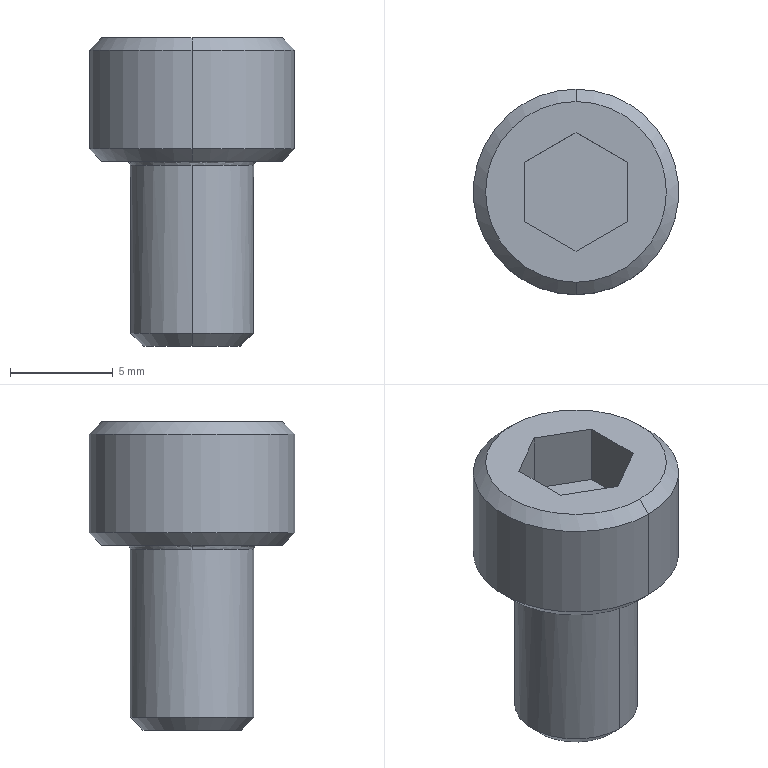Component | SolidWorks | TR-20x75-S-GN-1 (0)-3_5-1 | 1 solid | 22 faces | box 10 x 10 x 15 mm | volume 647 mm3 | plane 10 | cone 6 | cylinder 4 | spline 2 | commonest cylinder face diameters 6 x2 10 x2
STEP:
#1=COLOUR_RGB('',0.7922,0.8196,0.9333);
#2=FILL_AREA_STYLE_COLOUR('',#1);
#3=FILL_AREA_STYLE('',(#2));
#4=SURFACE_STYLE_FILL_AREA(#3);
#5=SURFACE_SIDE_STYLE('',(#4));
#6=SURFACE_STYLE_USAGE(.BOTH.,#5);
#7=PRESENTATION_STYLE_ASSIGNMENT((#6));
#8=CARTESIAN_POINT('',(7.52,25.197,0.4055));
#9=VERTEX_POINT('',#8);
#10=CARTESIAN_POINT('',(7.638,25.315,0.4055));
#11=VERTEX_POINT('',#10);
#12=CARTESIAN_POINT('',(7.638,25.197,0.4055));
#13=DIRECTION('',(-0.,0.,-1.));
#14=DIRECTION('',(0.,-1.,-0.));
#15=AXIS2_PLACEMENT_3D('',#12,#13,#14);
#16=CIRCLE('',#15,0.1181);
#17=EDGE_CURVE('',#9,#11,#16,.T.);
#18=ORIENTED_EDGE('',*,*,#17,.F.);
#19=CARTESIAN_POINT('',(7.512,25.197,0.4134));
#20=VERTEX_POINT('',#19);
#21=CARTESIAN_POINT('',(7.512,25.197,0.4055));
#22=DIRECTION('',(-0.,-1.,-0.));
#23=DIRECTION('',(-1.,0.,0.));
#24=AXIS2_PLACEMENT_3D('',#21,#22,#23);
#25=CIRCLE('',#24,0.007874);
#26=EDGE_CURVE('',#9,#20,#25,.T.);
#27=ORIENTED_EDGE('',*,*,#26,.T.);
#28=CARTESIAN_POINT('',(7.638,25.323,0.4134));
#29=VERTEX_POINT('',#28);
#30=CARTESIAN_POINT('',(7.638,25.323,0.4134));
#31=CARTESIAN_POINT('',(7.63,25.323,0.4134));
#32=CARTESIAN_POINT('',(7.618,25.322,0.4134));
#33=CARTESIAN_POINT('',(7.605,25.319,0.4134));
#34=CARTESIAN_POINT('',(7.598,25.316,0.4134));
#35=CARTESIAN_POINT('',(7.595,25.315,0.4134));
#36=CARTESIAN_POINT('',(7.593,25.315,0.4134));
#37=CARTESIAN_POINT('',(7.592,25.314,0.4134));
#38=CARTESIAN_POINT('',(7.575,25.308,0.4134));
#39=CARTESIAN_POINT('',(7.561,25.298,0.4134));
#40=CARTESIAN_POINT('',(7.543,25.28,0.4134));
#41=CARTESIAN_POINT('',(7.534,25.27,0.4134));
#42=CARTESIAN_POINT('',(7.527,25.257,0.4134));
#43=CARTESIAN_POINT('',(7.524,25.25,0.4134));
#44=CARTESIAN_POINT('',(7.522,25.247,0.4134));
#45=CARTESIAN_POINT('',(7.521,25.245,0.4134));
#46=CARTESIAN_POINT('',(7.521,25.244,0.4134));
#47=CARTESIAN_POINT('',(7.515,25.228,0.4134));
#48=CARTESIAN_POINT('',(7.512,25.213,0.4134));
#49=CARTESIAN_POINT('',(7.512,25.197,0.4134));
#50=B_SPLINE_CURVE_WITH_KNOTS('',3,(#30,#31,#32,#33,#34,#35,#36,#37,#38,#39,#40,#41,#42,#43,#44,#45,#46,#47,#48,#49),.UNSPECIFIED.,.F.,.F.,(4,1,1,1,2,2,2,1,1,1,2,2,4),(0.,0.125,0.1875,0.2188,0.2344,0.25,0.5,0.625,0.6875,0.7188,0.7344,0.75,1.),.UNSPECIFIED.);
#51=EDGE_CURVE('',#29,#20,#50,.T.);
#52=ORIENTED_EDGE('',*,*,#51,.F.);
#53=CARTESIAN_POINT('',(7.764,25.197,0.4134));
#54=VERTEX_POINT('',#53);
#55=CARTESIAN_POINT('',(7.764,25.197,0.4134));
#56=CARTESIAN_POINT('',(7.764,25.205,0.4134));
#57=CARTESIAN_POINT('',(7.763,25.217,0.4134));
#58=CARTESIAN_POINT('',(7.759,25.23,0.4134));
#59=CARTESIAN_POINT('',(7.757,25.237,0.4134));
#60=CARTESIAN_POINT('',(7.756,25.239,0.4134));
#61=CARTESIAN_POINT('',(7.756,25.241,0.4134));
#62=CARTESIAN_POINT('',(7.755,25.242,0.4134));
#63=CARTESIAN_POINT('',(7.749,25.259,0.4134));
#64=CARTESIAN_POINT('',(7.739,25.274,0.4134));
#65=CARTESIAN_POINT('',(7.721,25.292,0.4134));
#66=CARTESIAN_POINT('',(7.711,25.3,0.4134));
#67=CARTESIAN_POINT('',(7.698,25.308,0.4134));
#68=CARTESIAN_POINT('',(7.691,25.311,0.4134));
#69=CARTESIAN_POINT('',(7.688,25.312,0.4134));
#70=CARTESIAN_POINT('',(7.686,25.313,0.4134));
#71=CARTESIAN_POINT('',(7.685,25.314,0.4134));
#72=CARTESIAN_POINT('',(7.669,25.32,0.4134));
#73=CARTESIAN_POINT('',(7.654,25.323,0.4134));
#74=CARTESIAN_POINT('',(7.638,25.323,0.4134));
#75=B_SPLINE_CURVE_WITH_KNOTS('',3,(#55,#56,#57,#58,#59,#60,#61,#62,#63,#64,#65,#66,#67,#68,#69,#70,#71,#72,#73,#74),.UNSPECIFIED.,.F.,.F.,(4,1,1,1,2,2,2,1,1,1,2,2,4),(0.,0.125,0.1875,0.2187,0.2344,0.25,0.5,0.625,0.6875,0.7188,0.7344,0.75,1.),.UNSPECIFIED.);
#76=EDGE_CURVE('',#54,#29,#75,.T.);
#77=ORIENTED_EDGE('',*,*,#76,.F.);
#78=CARTESIAN_POINT('',(7.756,25.197,0.4055));
#79=VERTEX_POINT('',#78);
#80=CARTESIAN_POINT('',(7.764,25.197,0.4055));
#81=DIRECTION('',(0.,1.,0.));
#82=DIRECTION('',(1.,0.,0.));
#83=AXIS2_PLACEMENT_3D('',#80,#81,#82);
#84=CIRCLE('',#83,0.007874);
#85=EDGE_CURVE('',#79,#54,#84,.T.);
#86=ORIENTED_EDGE('',*,*,#85,.F.);
#87=CARTESIAN_POINT('',(7.638,25.197,0.4055));
#88=DIRECTION('',(-0.,0.,-1.));
#89=DIRECTION('',(0.,-1.,-0.));
#90=AXIS2_PLACEMENT_3D('',#87,#88,#89);
#91=CIRCLE('',#90,0.1181);
#92=EDGE_CURVE('',#11,#79,#91,.T.);
#93=ORIENTED_EDGE('',*,*,#92,.F.);
#94=EDGE_LOOP('',(#18,#27,#52,#77,#86,#93));
#95=FACE_OUTER_BOUND('',#94,.T.);
#96=CARTESIAN_POINT('',(7.756,25.197,0.4055));
#97=CARTESIAN_POINT('',(7.756,25.433,0.4055));
#98=CARTESIAN_POINT('',(7.52,25.433,0.4055));
#99=CARTESIAN_POINT('',(7.52,25.197,0.4055));
#100=CARTESIAN_POINT('',(7.756,25.197,0.4101));
#101=CARTESIAN_POINT('',(7.756,25.433,0.4101));
#102=CARTESIAN_POINT('',(7.52,25.433,0.4101));
#103=CARTESIAN_POINT('',(7.52,25.197,0.4101));
#104=CARTESIAN_POINT('',(7.759,25.197,0.4134));
#105=CARTESIAN_POINT('',(7.759,25.44,0.4134));
#106=CARTESIAN_POINT('',(7.516,25.44,0.4134));
#107=CARTESIAN_POINT('',(7.516,25.197,0.4134));
#108=CARTESIAN_POINT('',(7.764,25.197,0.4134));
#109=CARTESIAN_POINT('',(7.764,25.449,0.4134));
#110=CARTESIAN_POINT('',(7.512,25.449,0.4134));
#111=CARTESIAN_POINT('',(7.512,25.197,0.4134));
#112=(BOUNDED_SURFACE()B_SPLINE_SURFACE(3,3,((#96,#97,#98,#99),(#100,#101,#102,#103),(#104,#105,#106,#107),(#108,#109,#110,#111)),.UNSPECIFIED.,.F.,.F.,.T.)B_SPLINE_SURFACE_WITH_KNOTS((4,4),(4,4),(0.,1.),(0.,1.),.UNSPECIFIED.)GEOMETRIC_REPRESENTATION_ITEM()RATIONAL_B_SPLINE_SURFACE(((1.,0.3333,0.3333,1.),(0.8047,0.2682,0.2682,0.8047),(0.8047,0.2682,0.2682,0.8047),(1.,0.3333,0.3333,1.)))REPRESENTATION_ITEM('')SURFACE());
#113=ADVANCED_FACE('',(#95),#112,.F.);
#114=CARTESIAN_POINT('',(7.638,25.079,0.4055));
#115=VERTEX_POINT('',#114);
#116=CARTESIAN_POINT('',(7.638,25.197,0.4055));
#117=DIRECTION('',(-0.,0.,-1.));
#118=DIRECTION('',(0.,-1.,-0.));
#119=AXIS2_PLACEMENT_3D('',#116,#117,#118);
#120=CIRCLE('',#119,0.1181);
#121=EDGE_CURVE('',#115,#9,#120,.T.);
#122=ORIENTED_EDGE('',*,*,#121,.T.);
#123=ORIENTED_EDGE('',*,*,#17,.T.);
#124=CARTESIAN_POINT('',(7.638,25.315,0.08321));
#125=VERTEX_POINT('',#124);
#126=CARTESIAN_POINT('',(7.638,25.315,0.2444));
#127=DIRECTION('',(-0.,0.,-1.));
#128=VECTOR('',#127,39.37);
#129=LINE('',#126,#128);
#130=EDGE_CURVE('',#11,#125,#129,.T.);
#131=ORIENTED_EDGE('',*,*,#130,.T.);
#132=CARTESIAN_POINT('',(7.638,25.079,0.08321));
#133=VERTEX_POINT('',#132);
#134=CARTESIAN_POINT('',(7.638,25.197,0.08321));
#135=DIRECTION('',(0.,-0.,1.));
#136=DIRECTION('',(0.,-1.,-0.));
#137=AXIS2_PLACEMENT_3D('',#134,#135,#136);
#138=CIRCLE('',#137,0.1181);
#139=EDGE_CURVE('',#125,#133,#138,.T.);
#140=ORIENTED_EDGE('',*,*,#139,.T.);
#141=CARTESIAN_POINT('',(7.638,25.079,0.2444));
#142=DIRECTION('',(-0.,0.,-1.));
#143=VECTOR('',#142,39.37);
#144=LINE('',#141,#143);
#145=EDGE_CURVE('',#115,#133,#144,.T.);
#146=ORIENTED_EDGE('',*,*,#145,.F.);
#147=EDGE_LOOP('',(#122,#123,#131,#140,#146));
#148=FACE_OUTER_BOUND('',#147,.T.);
#149=CARTESIAN_POINT('',(7.638,25.197,0.2444));
#150=DIRECTION('',(-0.,0.,-1.));
#151=DIRECTION('',(0.,-1.,-0.));
#152=AXIS2_PLACEMENT_3D('',#149,#150,#151);
#153=CYLINDRICAL_SURFACE('',#152,0.1181);
#154=ADVANCED_FACE('',(#148),#153,.T.);
#155=CARTESIAN_POINT('',(7.638,25.291,0.05906));
#156=VERTEX_POINT('',#155);
#157=CARTESIAN_POINT('',(7.638,25.103,0.05906));
#158=VERTEX_POINT('',#157);
#159=CARTESIAN_POINT('',(7.638,25.197,0.05906));
#160=DIRECTION('',(0.,-0.,1.));
#161=DIRECTION('',(0.,1.,0.));
#162=AXIS2_PLACEMENT_3D('',#159,#160,#161);
#163=CIRCLE('',#162,0.09396);
#164=EDGE_CURVE('',#156,#158,#163,.T.);
#165=ORIENTED_EDGE('',*,*,#164,.T.);
#166=CARTESIAN_POINT('',(7.638,25.079,0.08321));
#167=DIRECTION('',(0.,-0.7071,0.7071));
#168=VECTOR('',#167,39.37);
#169=LINE('',#166,#168);
#170=EDGE_CURVE('',#158,#133,#169,.T.);
#171=ORIENTED_EDGE('',*,*,#170,.T.);
#172=ORIENTED_EDGE('',*,*,#139,.F.);
#173=CARTESIAN_POINT('',(7.638,25.315,0.08321));
#174=DIRECTION('',(0.,0.7071,0.7071));
#175=VECTOR('',#174,39.37);
#176=LINE('',#173,#175);
#177=EDGE_CURVE('',#156,#125,#176,.T.);
#178=ORIENTED_EDGE('',*,*,#177,.F.);
#179=EDGE_LOOP('',(#165,#171,#172,#178));
#180=FACE_OUTER_BOUND('',#179,.T.);
#181=CARTESIAN_POINT('',(7.638,25.197,0.08321));
#182=DIRECTION('',(0.,-0.,1.));
#183=DIRECTION('',(0.,1.,0.));
#184=AXIS2_PLACEMENT_3D('',#181,#182,#183);
#185=CONICAL_SURFACE('',#184,0.1181,0.7854);
#186=ADVANCED_FACE('',(#180),#185,.T.);
#187=CARTESIAN_POINT('',(7.638,25.024,0.4134));
#188=VERTEX_POINT('',#187);
#189=CARTESIAN_POINT('',(7.638,25.37,0.4134));
#190=VERTEX_POINT('',#189);
#191=CARTESIAN_POINT('',(7.638,25.197,0.4134));
#192=DIRECTION('',(-0.,0.,-1.));
#193=DIRECTION('',(0.,1.,0.));
#194=AXIS2_PLACEMENT_3D('',#191,#192,#193);
#195=CIRCLE('',#194,0.1732);
#196=EDGE_CURVE('',#188,#190,#195,.T.);
#197=ORIENTED_EDGE('',*,*,#196,.F.);
#198=CARTESIAN_POINT('',(7.638,25.,0.437));
#199=VERTEX_POINT('',#198);
#200=CARTESIAN_POINT('',(7.638,25.,0.437));
#201=DIRECTION('',(0.,-0.7071,0.7071));
#202=VECTOR('',#201,39.37);
#203=LINE('',#200,#202);
#204=EDGE_CURVE('',#188,#199,#203,.T.);
#205=ORIENTED_EDGE('',*,*,#204,.T.);
#206=CARTESIAN_POINT('',(7.638,25.394,0.437));
#207=VERTEX_POINT('',#206);
#208=CARTESIAN_POINT('',(7.638,25.197,0.437));
#209=DIRECTION('',(-0.,0.,-1.));
#210=DIRECTION('',(0.,1.,0.));
#211=AXIS2_PLACEMENT_3D('',#208,#209,#210);
#212=CIRCLE('',#211,0.1969);
#213=EDGE_CURVE('',#199,#207,#212,.T.);
#214=ORIENTED_EDGE('',*,*,#213,.T.);
#215=CARTESIAN_POINT('',(7.638,25.394,0.437));
#216=DIRECTION('',(0.,0.7071,0.7071));
#217=VECTOR('',#216,39.37);
#218=LINE('',#215,#217);
#219=EDGE_CURVE('',#190,#207,#218,.T.);
#220=ORIENTED_EDGE('',*,*,#219,.F.);
#221=EDGE_LOOP('',(#197,#205,#214,#220));
#222=FACE_OUTER_BOUND('',#221,.T.);
#223=CARTESIAN_POINT('',(7.638,25.197,0.437));
#224=DIRECTION('',(0.,-0.,1.));
#225=DIRECTION('',(0.,1.,0.));
#226=AXIS2_PLACEMENT_3D('',#223,#224,#225);
#227=CONICAL_SURFACE('',#226,0.1969,0.7854);
#228=ADVANCED_FACE('',(#222),#227,.T.);
#229=CARTESIAN_POINT('',(7.638,25.,0.626));
#230=VERTEX_POINT('',#229);
#231=CARTESIAN_POINT('',(7.638,25.394,0.626));
#232=VERTEX_POINT('',#231);
#233=CARTESIAN_POINT('',(7.638,25.197,0.626));
#234=DIRECTION('',(-0.,0.,-1.));
#235=DIRECTION('',(0.,-1.,-0.));
#236=AXIS2_PLACEMENT_3D('',#233,#234,#235);
#237=CIRCLE('',#236,0.1969);
#238=EDGE_CURVE('',#230,#232,#237,.T.);
#239=ORIENTED_EDGE('',*,*,#238,.T.);
#240=CARTESIAN_POINT('',(7.638,25.394,0.5315));
#241=DIRECTION('',(-0.,0.,-1.));
#242=VECTOR('',#241,39.37);
#243=LINE('',#240,#242);
#244=EDGE_CURVE('',#232,#207,#243,.T.);
#245=ORIENTED_EDGE('',*,*,#244,.T.);
#246=ORIENTED_EDGE('',*,*,#213,.F.);
#247=CARTESIAN_POINT('',(7.638,25.,0.5315));
#248=DIRECTION('',(-0.,0.,-1.));
#249=VECTOR('',#248,39.37);
#250=LINE('',#247,#249);
#251=EDGE_CURVE('',#230,#199,#250,.T.);
#252=ORIENTED_EDGE('',*,*,#251,.F.);
#253=EDGE_LOOP('',(#239,#245,#246,#252));
#254=FACE_OUTER_BOUND('',#253,.T.);
#255=CARTESIAN_POINT('',(7.638,25.197,0.5315));
#256=DIRECTION('',(-0.,0.,-1.));
#257=DIRECTION('',(0.,-1.,-0.));
#258=AXIS2_PLACEMENT_3D('',#255,#256,#257);
#259=CYLINDRICAL_SURFACE('',#258,0.1969);
#260=ADVANCED_FACE('',(#254),#259,.T.);
#261=CARTESIAN_POINT('',(7.638,25.024,0.6496));
#262=VERTEX_POINT('',#261);
#263=CARTESIAN_POINT('',(7.638,25.37,0.6496));
#264=VERTEX_POINT('',#263);
#265=CARTESIAN_POINT('',(7.638,25.197,0.6496));
#266=DIRECTION('',(-0.,0.,-1.));
#267=DIRECTION('',(0.,-1.,-0.));
#268=AXIS2_PLACEMENT_3D('',#265,#266,#267);
#269=CIRCLE('',#268,0.1732);
#270=EDGE_CURVE('',#262,#264,#269,.T.);
#271=ORIENTED_EDGE('',*,*,#270,.T.);
#272=CARTESIAN_POINT('',(7.638,25.394,0.626));
#273=DIRECTION('',(-0.,0.7071,-0.7071));
#274=VECTOR('',#273,39.37);
#275=LINE('',#272,#274);
#276=EDGE_CURVE('',#264,#232,#275,.T.);
#277=ORIENTED_EDGE('',*,*,#276,.T.);
#278=ORIENTED_EDGE('',*,*,#238,.F.);
#279=CARTESIAN_POINT('',(7.638,25.,0.626));
#280=DIRECTION('',(-0.,-0.7071,-0.7071));
#281=VECTOR('',#280,39.37);
#282=LINE('',#279,#281);
#283=EDGE_CURVE('',#262,#230,#282,.T.);
#284=ORIENTED_EDGE('',*,*,#283,.F.);
#285=EDGE_LOOP('',(#271,#277,#278,#284));
#286=FACE_OUTER_BOUND('',#285,.T.);
#287=CARTESIAN_POINT('',(7.638,25.197,0.626));
#288=DIRECTION('',(-0.,0.,-1.));
#289=DIRECTION('',(0.,-1.,-0.));
#290=AXIS2_PLACEMENT_3D('',#287,#288,#289);
#291=CONICAL_SURFACE('',#290,0.1969,0.7854);
#292=ADVANCED_FACE('',(#286),#291,.T.);
#293=ORIENTED_EDGE('',*,*,#130,.F.);
#294=ORIENTED_EDGE('',*,*,#92,.T.);
#295=CARTESIAN_POINT('',(7.638,25.197,0.4055));
#296=DIRECTION('',(-0.,0.,-1.));
#297=DIRECTION('',(0.,-1.,-0.));
#298=AXIS2_PLACEMENT_3D('',#295,#296,#297);
#299=CIRCLE('',#298,0.1181);
#300=EDGE_CURVE('',#79,#115,#299,.T.);
#301=ORIENTED_EDGE('',*,*,#300,.T.);
#302=ORIENTED_EDGE('',*,*,#145,.T.);
#303=CARTESIAN_POINT('',(7.638,25.197,0.08321));
#304=DIRECTION('',(0.,-0.,1.));
#305=DIRECTION('',(0.,-1.,-0.));
#306=AXIS2_PLACEMENT_3D('',#303,#304,#305);
#307=CIRCLE('',#306,0.1181);
#308=EDGE_CURVE('',#133,#125,#307,.T.);
#309=ORIENTED_EDGE('',*,*,#308,.T.);
#310=EDGE_LOOP('',(#293,#294,#301,#302,#309));
#311=FACE_OUTER_BOUND('',#310,.T.);
#312=CARTESIAN_POINT('',(7.638,25.197,0.2444));
#313=DIRECTION('',(-0.,0.,-1.));
#314=DIRECTION('',(0.,-1.,-0.));
#315=AXIS2_PLACEMENT_3D('',#312,#313,#314);
#316=CYLINDRICAL_SURFACE('',#315,0.1181);
#317=ADVANCED_FACE('',(#311),#316,.T.);
#318=ORIENTED_EDGE('',*,*,#26,.F.);
#319=ORIENTED_EDGE('',*,*,#121,.F.);
#320=ORIENTED_EDGE('',*,*,#300,.F.);
#321=ORIENTED_EDGE('',*,*,#85,.T.);
#322=CARTESIAN_POINT('',(7.512,25.197,0.4134));
#323=CARTESIAN_POINT('',(7.512,25.189,0.4134));
#324=CARTESIAN_POINT('',(7.513,25.177,0.4134));
#325=CARTESIAN_POINT('',(7.516,25.164,0.4134));
#326=CARTESIAN_POINT('',(7.518,25.157,0.4134));
#327=CARTESIAN_POINT('',(7.519,25.154,0.4134));
#328=CARTESIAN_POINT('',(7.52,25.152,0.4134));
#329=CARTESIAN_POINT('',(7.52,25.151,0.4134));
#330=CARTESIAN_POINT('',(7.527,25.134,0.4134));
#331=CARTESIAN_POINT('',(7.536,25.12,0.4134));
#332=CARTESIAN_POINT('',(7.555,25.102,0.4134));
#333=CARTESIAN_POINT('',(7.565,25.094,0.4134));
#334=CARTESIAN_POINT('',(7.578,25.086,0.4134));
#335=CARTESIAN_POINT('',(7.584,25.083,0.4134));
#336=CARTESIAN_POINT('',(7.587,25.081,0.4134));
#337=CARTESIAN_POINT('',(7.589,25.081,0.4134));
#338=CARTESIAN_POINT('',(7.59,25.08,0.4134));
#339=CARTESIAN_POINT('',(7.606,25.074,0.4134));
#340=CARTESIAN_POINT('',(7.622,25.071,0.4134));
#341=CARTESIAN_POINT('',(7.646,25.071,0.4134));
#342=CARTESIAN_POINT('',(7.658,25.072,0.4134));
#343=CARTESIAN_POINT('',(7.671,25.075,0.4134));
#344=CARTESIAN_POINT('',(7.678,25.077,0.4134));
#345=CARTESIAN_POINT('',(7.68,25.078,0.4134));
#346=CARTESIAN_POINT('',(7.682,25.079,0.4134));
#347=CARTESIAN_POINT('',(7.683,25.079,0.4134));
#348=CARTESIAN_POINT('',(7.7,25.086,0.4134));
#349=CARTESIAN_POINT('',(7.715,25.095,0.4134));
#350=CARTESIAN_POINT('',(7.733,25.114,0.4134));
#351=CARTESIAN_POINT('',(7.741,25.124,0.4134));
#352=CARTESIAN_POINT('',(7.749,25.137,0.4134));
#353=CARTESIAN_POINT('',(7.752,25.144,0.4134));
#354=CARTESIAN_POINT('',(7.753,25.146,0.4134));
#355=CARTESIAN_POINT('',(7.754,25.148,0.4134));
#356=CARTESIAN_POINT('',(7.755,25.15,0.4134));
#357=CARTESIAN_POINT('',(7.761,25.165,0.4134));
#358=CARTESIAN_POINT('',(7.764,25.181,0.4134));
#359=CARTESIAN_POINT('',(7.764,25.197,0.4134));
#360=B_SPLINE_CURVE_WITH_KNOTS('',3,(#322,#323,#324,#325,#326,#327,#328,#329,#330,#331,#332,#333,#334,#335,#336,#337,#338,#339,#340,#341,#342,#343,#344,#345,#346,#347,#348,#349,#350,#351,#352,#353,#354,#355,#356,#357,#358,#359),.UNSPECIFIED.,.F.,.F.,(4,1,1,1,2,2,2,1,1,1,2,2,2,1,1,1,2,2,2,1,1,1,2,2,4),(0.,0.0625,0.09375,0.1094,0.1172,0.125,0.25,0.3125,0.3437,0.3594,0.3672,0.375,0.5,0.5625,0.5937,0.6094,0.6172,0.625,0.75,0.8125,0.8437,0.8594,0.8672,0.875,1.),.UNSPECIFIED.);
#361=EDGE_CURVE('',#20,#54,#360,.T.);
#362=ORIENTED_EDGE('',*,*,#361,.F.);
#363=EDGE_LOOP('',(#318,#319,#320,#321,#362));
#364=FACE_OUTER_BOUND('',#363,.T.);
#365=CARTESIAN_POINT('',(7.52,25.197,0.4055));
#366=CARTESIAN_POINT('',(7.52,24.961,0.4055));
#367=CARTESIAN_POINT('',(7.756,24.961,0.4055));
#368=CARTESIAN_POINT('',(7.756,25.197,0.4055));
#369=CARTESIAN_POINT('',(7.52,25.197,0.4101));
#370=CARTESIAN_POINT('',(7.52,24.961,0.4101));
#371=CARTESIAN_POINT('',(7.756,24.961,0.4101));
#372=CARTESIAN_POINT('',(7.756,25.197,0.4101));
#373=CARTESIAN_POINT('',(7.516,25.197,0.4134));
#374=CARTESIAN_POINT('',(7.516,24.954,0.4134));
#375=CARTESIAN_POINT('',(7.759,24.954,0.4134));
#376=CARTESIAN_POINT('',(7.759,25.197,0.4134));
#377=CARTESIAN_POINT('',(7.512,25.197,0.4134));
#378=CARTESIAN_POINT('',(7.512,24.945,0.4134));
#379=CARTESIAN_POINT('',(7.764,24.945,0.4134));
#380=CARTESIAN_POINT('',(7.764,25.197,0.4134));
#381=(BOUNDED_SURFACE()B_SPLINE_SURFACE(3,3,((#365,#366,#367,#368),(#369,#370,#371,#372),(#373,#374,#375,#376),(#377,#378,#379,#380)),.UNSPECIFIED.,.F.,.F.,.F.)B_SPLINE_SURFACE_WITH_KNOTS((4,4),(4,4),(0.,1.),(0.,1.),.UNSPECIFIED.)GEOMETRIC_REPRESENTATION_ITEM()RATIONAL_B_SPLINE_SURFACE(((1.,0.3333,0.3333,1.),(0.8047,0.2682,0.2682,0.8047),(0.8047,0.2682,0.2682,0.8047),(1.,0.3333,0.3333,1.)))REPRESENTATION_ITEM('')SURFACE());
#382=ADVANCED_FACE('',(#364),#381,.F.);
#383=ORIENTED_EDGE('',*,*,#170,.F.);
#384=CARTESIAN_POINT('',(7.638,25.197,0.05906));
#385=DIRECTION('',(0.,-0.,1.));
#386=DIRECTION('',(0.,1.,0.));
#387=AXIS2_PLACEMENT_3D('',#384,#385,#386);
#388=CIRCLE('',#387,0.09396);
#389=EDGE_CURVE('',#158,#156,#388,.T.);
#390=ORIENTED_EDGE('',*,*,#389,.T.);
#391=ORIENTED_EDGE('',*,*,#177,.T.);
#392=ORIENTED_EDGE('',*,*,#308,.F.);
#393=EDGE_LOOP('',(#383,#390,#391,#392));
#394=FACE_OUTER_BOUND('',#393,.T.);
#395=CARTESIAN_POINT('',(7.638,25.197,0.08321));
#396=DIRECTION('',(0.,-0.,1.));
#397=DIRECTION('',(0.,1.,0.));
#398=AXIS2_PLACEMENT_3D('',#395,#396,#397);
#399=CONICAL_SURFACE('',#398,0.1181,0.7854);
#400=ADVANCED_FACE('',(#394),#399,.T.);
#401=ORIENTED_EDGE('',*,*,#361,.T.);
#402=ORIENTED_EDGE('',*,*,#76,.T.);
#403=ORIENTED_EDGE('',*,*,#51,.T.);
#404=EDGE_LOOP('',(#401,#402,#403));
#405=FACE_BOUND('',#404,.T.);
#406=CARTESIAN_POINT('',(7.638,25.197,0.4134));
#407=DIRECTION('',(-0.,0.,-1.));
#408=DIRECTION('',(0.,1.,0.));
#409=AXIS2_PLACEMENT_3D('',#406,#407,#408);
#410=CIRCLE('',#409,0.1732);
#411=EDGE_CURVE('',#190,#188,#410,.T.);
#412=ORIENTED_EDGE('',*,*,#411,.T.);
#413=ORIENTED_EDGE('',*,*,#196,.T.);
#414=EDGE_LOOP('',(#412,#413));
#415=FACE_OUTER_BOUND('',#414,.T.);
#416=CARTESIAN_POINT('',(7.638,25.346,0.4134));
#417=DIRECTION('',(-0.,0.,-1.));
#418=DIRECTION('',(-0.,-1.,-0.));
#419=AXIS2_PLACEMENT_3D('',#416,#417,#418);
#420=PLANE('',#419);
#421=ADVANCED_FACE('',(#405,#415),#420,.T.);
#422=ORIENTED_EDGE('',*,*,#164,.F.);
#423=ORIENTED_EDGE('',*,*,#389,.F.);
#424=EDGE_LOOP('',(#422,#423));
#425=FACE_OUTER_BOUND('',#424,.T.);
#426=CARTESIAN_POINT('',(7.638,25.244,0.05906));
#427=DIRECTION('',(-0.,0.,-1.));
#428=DIRECTION('',(-0.,-1.,-0.));
#429=AXIS2_PLACEMENT_3D('',#426,#427,#428);
#430=PLANE('',#429);
#431=ADVANCED_FACE('',(#425),#430,.T.);
#432=ORIENTED_EDGE('',*,*,#204,.F.);
#433=ORIENTED_EDGE('',*,*,#411,.F.);
#434=ORIENTED_EDGE('',*,*,#219,.T.);
#435=CARTESIAN_POINT('',(7.638,25.197,0.437));
#436=DIRECTION('',(-0.,0.,-1.));
#437=DIRECTION('',(0.,1.,0.));
#438=AXIS2_PLACEMENT_3D('',#435,#436,#437);
#439=CIRCLE('',#438,0.1969);
#440=EDGE_CURVE('',#207,#199,#439,.T.);
#441=ORIENTED_EDGE('',*,*,#440,.T.);
#442=EDGE_LOOP('',(#432,#433,#434,#441));
#443=FACE_OUTER_BOUND('',#442,.T.);
#444=CARTESIAN_POINT('',(7.638,25.197,0.437));
#445=DIRECTION('',(0.,-0.,1.));
#446=DIRECTION('',(0.,1.,0.));
#447=AXIS2_PLACEMENT_3D('',#444,#445,#446);
#448=CONICAL_SURFACE('',#447,0.1969,0.7854);
#449=ADVANCED_FACE('',(#443),#448,.T.);
#450=ORIENTED_EDGE('',*,*,#244,.F.);
#451=CARTESIAN_POINT('',(7.638,25.197,0.626));
#452=DIRECTION('',(-0.,0.,-1.));
#453=DIRECTION('',(0.,-1.,-0.));
#454=AXIS2_PLACEMENT_3D('',#451,#452,#453);
#455=CIRCLE('',#454,0.1969);
#456=EDGE_CURVE('',#232,#230,#455,.T.);
#457=ORIENTED_EDGE('',*,*,#456,.T.);
#458=ORIENTED_EDGE('',*,*,#251,.T.);
#459=ORIENTED_EDGE('',*,*,#440,.F.);
#460=EDGE_LOOP('',(#450,#457,#458,#459));
#461=FACE_OUTER_BOUND('',#460,.T.);
#462=CARTESIAN_POINT('',(7.638,25.197,0.5315));
#463=DIRECTION('',(-0.,0.,-1.));
#464=DIRECTION('',(0.,-1.,-0.));
#465=AXIS2_PLACEMENT_3D('',#462,#463,#464);
#466=CYLINDRICAL_SURFACE('',#465,0.1969);
#467=ADVANCED_FACE('',(#461),#466,.T.);
#468=ORIENTED_EDGE('',*,*,#276,.F.);
#469=CARTESIAN_POINT('',(7.638,25.197,0.6496));
#470=DIRECTION('',(-0.,0.,-1.));
#471=DIRECTION('',(0.,-1.,-0.));
#472=AXIS2_PLACEMENT_3D('',#469,#470,#471);
#473=CIRCLE('',#472,0.1732);
#474=EDGE_CURVE('',#264,#262,#473,.T.);
#475=ORIENTED_EDGE('',*,*,#474,.T.);
#476=ORIENTED_EDGE('',*,*,#283,.T.);
#477=ORIENTED_EDGE('',*,*,#456,.F.);
#478=EDGE_LOOP('',(#468,#475,#476,#477));
#479=FACE_OUTER_BOUND('',#478,.T.);
#480=CARTESIAN_POINT('',(7.638,25.197,0.626));
#481=DIRECTION('',(-0.,0.,-1.));
#482=DIRECTION('',(0.,-1.,-0.));
#483=AXIS2_PLACEMENT_3D('',#480,#481,#482);
#484=CONICAL_SURFACE('',#483,0.1969,0.7854);
#485=ADVANCED_FACE('',(#479),#484,.T.);
#486=ORIENTED_EDGE('',*,*,#270,.F.);
#487=ORIENTED_EDGE('',*,*,#474,.F.);
#488=EDGE_LOOP('',(#486,#487));
#489=FACE_OUTER_BOUND('',#488,.T.);
#490=CARTESIAN_POINT('',(7.539,25.14,0.6496));
#491=VERTEX_POINT('',#490);
#492=CARTESIAN_POINT('',(7.539,25.254,0.6496));
#493=VERTEX_POINT('',#492);
#494=CARTESIAN_POINT('',(7.539,25.283,0.6496));
#495=DIRECTION('',(0.,1.,0.));
#496=VECTOR('',#495,39.37);
#497=LINE('',#494,#496);
#498=EDGE_CURVE('',#491,#493,#497,.T.);
#499=ORIENTED_EDGE('',*,*,#498,.T.);
#500=CARTESIAN_POINT('',(7.638,25.311,0.6496));
#501=VERTEX_POINT('',#500);
#502=CARTESIAN_POINT('',(7.539,25.254,0.6496));
#503=DIRECTION('',(0.866,0.5,0.));
#504=VECTOR('',#503,39.37);
#505=LINE('',#502,#504);
#506=EDGE_CURVE('',#493,#501,#505,.T.);
#507=ORIENTED_EDGE('',*,*,#506,.T.);
#508=CARTESIAN_POINT('',(7.736,25.254,0.6496));
#509=VERTEX_POINT('',#508);
#510=CARTESIAN_POINT('',(7.638,25.311,0.6496));
#511=DIRECTION('',(0.866,-0.5,-0.));
#512=VECTOR('',#511,39.37);
#513=LINE('',#510,#512);
#514=EDGE_CURVE('',#501,#509,#513,.T.);
#515=ORIENTED_EDGE('',*,*,#514,.T.);
#516=CARTESIAN_POINT('',(7.736,25.14,0.6496));
#517=VERTEX_POINT('',#516);
#518=CARTESIAN_POINT('',(7.736,25.283,0.6496));
#519=DIRECTION('',(-0.,-1.,-0.));
#520=VECTOR('',#519,39.37);
#521=LINE('',#518,#520);
#522=EDGE_CURVE('',#509,#517,#521,.T.);
#523=ORIENTED_EDGE('',*,*,#522,.T.);
#524=CARTESIAN_POINT('',(7.638,25.083,0.6496));
#525=VERTEX_POINT('',#524);
#526=CARTESIAN_POINT('',(7.736,25.14,0.6496));
#527=DIRECTION('',(-0.866,-0.5,-0.));
#528=VECTOR('',#527,39.37);
#529=LINE('',#526,#528);
#530=EDGE_CURVE('',#517,#525,#529,.T.);
#531=ORIENTED_EDGE('',*,*,#530,.T.);
#532=CARTESIAN_POINT('',(7.638,25.083,0.6496));
#533=DIRECTION('',(-0.866,0.5,0.));
#534=VECTOR('',#533,39.37);
#535=LINE('',#532,#534);
#536=EDGE_CURVE('',#525,#491,#535,.T.);
#537=ORIENTED_EDGE('',*,*,#536,.T.);
#538=EDGE_LOOP('',(#499,#507,#515,#523,#531,#537));
#539=FACE_BOUND('',#538,.T.);
#540=CARTESIAN_POINT('',(7.638,25.283,0.6496));
#541=DIRECTION('',(0.,-0.,1.));
#542=DIRECTION('',(0.,1.,0.));
#543=AXIS2_PLACEMENT_3D('',#540,#541,#542);
#544=PLANE('',#543);
#545=ADVANCED_FACE('',(#489,#539),#544,.T.);
#546=CARTESIAN_POINT('',(7.638,25.311,0.5315));
#547=VERTEX_POINT('',#546);
#548=CARTESIAN_POINT('',(7.638,25.311,0.6496));
#549=DIRECTION('',(-0.,0.,-1.));
#550=VECTOR('',#549,39.37);
#551=LINE('',#548,#550);
#552=EDGE_CURVE('',#501,#547,#551,.T.);
#553=ORIENTED_EDGE('',*,*,#552,.F.);
#554=ORIENTED_EDGE('',*,*,#506,.F.);
#555=CARTESIAN_POINT('',(7.539,25.254,0.5315));
#556=VERTEX_POINT('',#555);
#557=CARTESIAN_POINT('',(7.539,25.254,0.6496));
#558=DIRECTION('',(0.,-0.,1.));
#559=VECTOR('',#558,39.37);
#560=LINE('',#557,#559);
#561=EDGE_CURVE('',#556,#493,#560,.T.);
#562=ORIENTED_EDGE('',*,*,#561,.F.);
#563=CARTESIAN_POINT('',(7.638,25.311,0.5315));
#564=DIRECTION('',(-0.866,-0.5,-0.));
#565=VECTOR('',#564,39.37);
#566=LINE('',#563,#565);
#567=EDGE_CURVE('',#547,#556,#566,.T.);
#568=ORIENTED_EDGE('',*,*,#567,.F.);
#569=EDGE_LOOP('',(#553,#554,#562,#568));
#570=FACE_OUTER_BOUND('',#569,.T.);
#571=CARTESIAN_POINT('',(7.638,25.311,0.6496));
#572=DIRECTION('',(-0.5,0.866,0.));
#573=DIRECTION('',(0.866,0.5,0.));
#574=AXIS2_PLACEMENT_3D('',#571,#572,#573);
#575=PLANE('',#574);
#576=ADVANCED_FACE('',(#570),#575,.F.);
#577=ORIENTED_EDGE('',*,*,#561,.T.);
#578=ORIENTED_EDGE('',*,*,#498,.F.);
#579=CARTESIAN_POINT('',(7.539,25.14,0.5315));
#580=VERTEX_POINT('',#579);
#581=CARTESIAN_POINT('',(7.539,25.14,0.6496));
#582=DIRECTION('',(0.,-0.,1.));
#583=VECTOR('',#582,39.37);
#584=LINE('',#581,#583);
#585=EDGE_CURVE('',#580,#491,#584,.T.);
#586=ORIENTED_EDGE('',*,*,#585,.F.);
#587=CARTESIAN_POINT('',(7.539,25.254,0.5315));
#588=DIRECTION('',(-0.,-1.,-0.));
#589=VECTOR('',#588,39.37);
#590=LINE('',#587,#589);
#591=EDGE_CURVE('',#556,#580,#590,.T.);
#592=ORIENTED_EDGE('',*,*,#591,.F.);
#593=EDGE_LOOP('',(#577,#578,#586,#592));
#594=FACE_OUTER_BOUND('',#593,.T.);
#595=CARTESIAN_POINT('',(7.539,25.254,0.6496));
#596=DIRECTION('',(-1.,0.,0.));
#597=DIRECTION('',(0.,1.,0.));
#598=AXIS2_PLACEMENT_3D('',#595,#596,#597);
#599=PLANE('',#598);
#600=ADVANCED_FACE('',(#594),#599,.F.);
#601=ORIENTED_EDGE('',*,*,#585,.T.);
#602=ORIENTED_EDGE('',*,*,#536,.F.);
#603=CARTESIAN_POINT('',(7.638,25.083,0.5315));
#604=VERTEX_POINT('',#603);
#605=CARTESIAN_POINT('',(7.638,25.083,0.6496));
#606=DIRECTION('',(0.,-0.,1.));
#607=VECTOR('',#606,39.37);
#608=LINE('',#605,#607);
#609=EDGE_CURVE('',#604,#525,#608,.T.);
#610=ORIENTED_EDGE('',*,*,#609,.F.);
#611=CARTESIAN_POINT('',(7.539,25.14,0.5315));
#612=DIRECTION('',(0.866,-0.5,-0.));
#613=VECTOR('',#612,39.37);
#614=LINE('',#611,#613);
#615=EDGE_CURVE('',#580,#604,#614,.T.);
#616=ORIENTED_EDGE('',*,*,#615,.F.);
#617=EDGE_LOOP('',(#601,#602,#610,#616));
#618=FACE_OUTER_BOUND('',#617,.T.);
#619=CARTESIAN_POINT('',(7.539,25.14,0.6496));
#620=DIRECTION('',(-0.5,-0.866,-0.));
#621=DIRECTION('',(-0.866,0.5,0.));
#622=AXIS2_PLACEMENT_3D('',#619,#620,#621);
#623=PLANE('',#622);
#624=ADVANCED_FACE('',(#618),#623,.F.);
#625=ORIENTED_EDGE('',*,*,#609,.T.);
#626=ORIENTED_EDGE('',*,*,#530,.F.);
#627=CARTESIAN_POINT('',(7.736,25.14,0.5315));
#628=VERTEX_POINT('',#627);
#629=CARTESIAN_POINT('',(7.736,25.14,0.6496));
#630=DIRECTION('',(0.,-0.,1.));
#631=VECTOR('',#630,39.37);
#632=LINE('',#629,#631);
#633=EDGE_CURVE('',#628,#517,#632,.T.);
#634=ORIENTED_EDGE('',*,*,#633,.F.);
#635=CARTESIAN_POINT('',(7.638,25.083,0.5315));
#636=DIRECTION('',(0.866,0.5,0.));
#637=VECTOR('',#636,39.37);
#638=LINE('',#635,#637);
#639=EDGE_CURVE('',#604,#628,#638,.T.);
#640=ORIENTED_EDGE('',*,*,#639,.F.);
#641=EDGE_LOOP('',(#625,#626,#634,#640));
#642=FACE_OUTER_BOUND('',#641,.T.);
#643=CARTESIAN_POINT('',(7.638,25.083,0.6496));
#644=DIRECTION('',(0.5,-0.866,-0.));
#645=DIRECTION('',(-0.866,-0.5,-0.));
#646=AXIS2_PLACEMENT_3D('',#643,#644,#645);
#647=PLANE('',#646);
#648=ADVANCED_FACE('',(#642),#647,.F.);
#649=ORIENTED_EDGE('',*,*,#633,.T.);
#650=ORIENTED_EDGE('',*,*,#522,.F.);
#651=CARTESIAN_POINT('',(7.736,25.254,0.5315));
#652=VERTEX_POINT('',#651);
#653=CARTESIAN_POINT('',(7.736,25.254,0.6496));
#654=DIRECTION('',(0.,-0.,1.));
#655=VECTOR('',#654,39.37);
#656=LINE('',#653,#655);
#657=EDGE_CURVE('',#652,#509,#656,.T.);
#658=ORIENTED_EDGE('',*,*,#657,.F.);
#659=CARTESIAN_POINT('',(7.736,25.14,0.5315));
#660=DIRECTION('',(0.,1.,0.));
#661=VECTOR('',#660,39.37);
#662=LINE('',#659,#661);
#663=EDGE_CURVE('',#628,#652,#662,.T.);
#664=ORIENTED_EDGE('',*,*,#663,.F.);
#665=EDGE_LOOP('',(#649,#650,#658,#664));
#666=FACE_OUTER_BOUND('',#665,.T.);
#667=CARTESIAN_POINT('',(7.736,25.14,0.6496));
#668=DIRECTION('',(1.,0.,-0.));
#669=DIRECTION('',(-0.,-1.,-0.));
#670=AXIS2_PLACEMENT_3D('',#667,#668,#669);
#671=PLANE('',#670);
#672=ADVANCED_FACE('',(#666),#671,.F.);
#673=ORIENTED_EDGE('',*,*,#657,.T.);
#674=ORIENTED_EDGE('',*,*,#514,.F.);
#675=ORIENTED_EDGE('',*,*,#552,.T.);
#676=CARTESIAN_POINT('',(7.736,25.254,0.5315));
#677=DIRECTION('',(-0.866,0.5,0.));
#678=VECTOR('',#677,39.37);
#679=LINE('',#676,#678);
#680=EDGE_CURVE('',#652,#547,#679,.T.);
#681=ORIENTED_EDGE('',*,*,#680,.F.);
#682=EDGE_LOOP('',(#673,#674,#675,#681));
#683=FACE_OUTER_BOUND('',#682,.T.);
#684=CARTESIAN_POINT('',(7.736,25.254,0.6496));
#685=DIRECTION('',(0.5,0.866,0.));
#686=DIRECTION('',(0.866,-0.5,-0.));
#687=AXIS2_PLACEMENT_3D('',#684,#685,#686);
#688=PLANE('',#687);
#689=ADVANCED_FACE('',(#683),#688,.F.);
#690=ORIENTED_EDGE('',*,*,#567,.T.);
#691=ORIENTED_EDGE('',*,*,#591,.T.);
#692=ORIENTED_EDGE('',*,*,#615,.T.);
#693=ORIENTED_EDGE('',*,*,#639,.T.);
#694=ORIENTED_EDGE('',*,*,#663,.T.);
#695=ORIENTED_EDGE('',*,*,#680,.T.);
#696=EDGE_LOOP('',(#690,#691,#692,#693,#694,#695));
#697=FACE_OUTER_BOUND('',#696,.T.);
#698=CARTESIAN_POINT('',(7.638,25.197,0.5315));
#699=DIRECTION('',(-0.,0.,-1.));
#700=DIRECTION('',(-0.,-1.,-0.));
#701=AXIS2_PLACEMENT_3D('',#698,#699,#700);
#702=PLANE('',#701);
#703=ADVANCED_FACE('',(#697),#702,.F.);
#704=CLOSED_SHELL('',(#113,#154,#186,#228,#260,#292,#317,#382,#400,#421,#431,#449,#467,#485,#545,#576,#600,#624,#648,#672,#689,#703));
#705=MANIFOLD_SOLID_BREP('',#704);
#706=STYLED_ITEM('',(#7),#705);
#707=PRESENTATION_LAYER_ASSIGNMENT('','',(#706));
#708=(LENGTH_UNIT()NAMED_UNIT(*)SI_UNIT($,.METRE.));
#709=LENGTH_MEASURE_WITH_UNIT(LENGTH_MEASURE(0.0254),#708);
#710=DIMENSIONAL_EXPONENTS(1.,0.,0.,0.,0.,0.,0.);
#711=(CONVERSION_BASED_UNIT('',#709)LENGTH_UNIT()NAMED_UNIT(#710));
#712=UNCERTAINTY_MEASURE_WITH_UNIT(LENGTH_MEASURE(0.00001),#711,'','');
#713=(NAMED_UNIT(*)PLANE_ANGLE_UNIT()SI_UNIT($,.RADIAN.));
#714=(NAMED_UNIT(*)SI_UNIT($,.STERADIAN.)SOLID_ANGLE_UNIT());
#715=(GEOMETRIC_REPRESENTATION_CONTEXT(3)GLOBAL_UNCERTAINTY_ASSIGNED_CONTEXT((#712))GLOBAL_UNIT_ASSIGNED_CONTEXT((#711,#713,#714))REPRESENTATION_CONTEXT('',''));
#716=MECHANICAL_DESIGN_GEOMETRIC_PRESENTATION_REPRESENTATION('',(#706),#715);
#717=CARTESIAN_POINT('',(0.,0.,0.));
#718=DIRECTION('',(0.,0.,1.));
#719=DIRECTION('',(1.,0.,0.));
#720=AXIS2_PLACEMENT_3D('',#717,#718,#719);
#721=(LENGTH_UNIT()NAMED_UNIT(*)SI_UNIT($,.METRE.));
#722=LENGTH_MEASURE_WITH_UNIT(LENGTH_MEASURE(0.0254),#721);
#723=DIMENSIONAL_EXPONENTS(1.,0.,0.,0.,0.,0.,0.);
#724=(CONVERSION_BASED_UNIT('',#722)LENGTH_UNIT()NAMED_UNIT(#723));
#725=UNCERTAINTY_MEASURE_WITH_UNIT(LENGTH_MEASURE(0.00001),#724,'','');
#726=(NAMED_UNIT(*)PLANE_ANGLE_UNIT()SI_UNIT($,.RADIAN.));
#727=(NAMED_UNIT(*)SI_UNIT($,.STERADIAN.)SOLID_ANGLE_UNIT());
#728=(GEOMETRIC_REPRESENTATION_CONTEXT(3)GLOBAL_UNCERTAINTY_ASSIGNED_CONTEXT((#725))GLOBAL_UNIT_ASSIGNED_CONTEXT((#724,#726,#727))REPRESENTATION_CONTEXT('',''));
#729=ADVANCED_BREP_SHAPE_REPRESENTATION('',(#705,#720),#728);